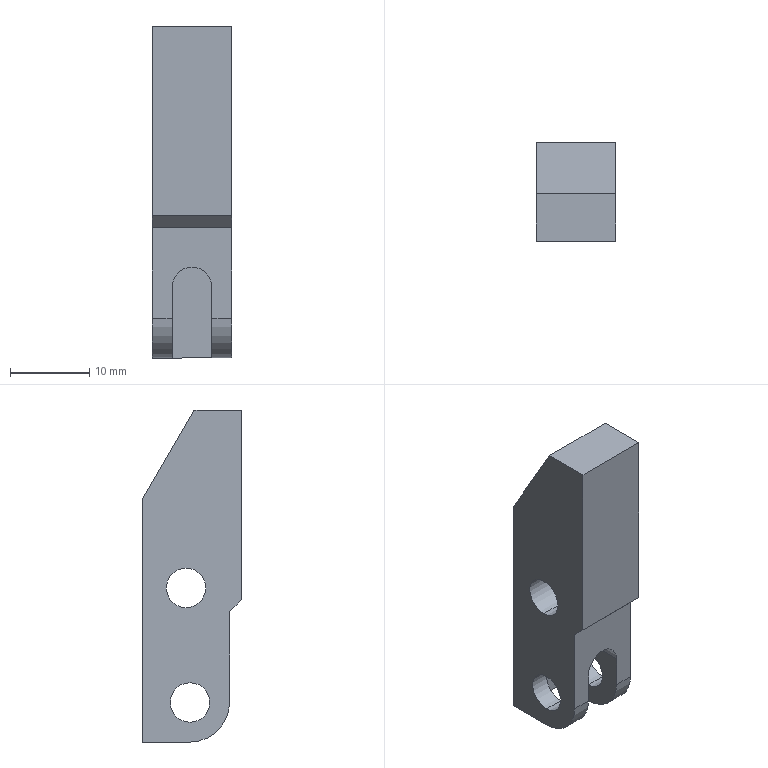Component | SolidWorks | LeverHydraulicRod22-1_HLKA-22_-1-1 | 1 solid | 21 faces | box 10 x 12.5 x 42 mm | volume 3756 mm3 | plane 12 | cylinder 9 | commonest cylinder face diameters 5 x7 10 x2
STEP:
#1=COLOUR_RGB('',0.7922,0.8196,0.9333);
#2=FILL_AREA_STYLE_COLOUR('',#1);
#3=FILL_AREA_STYLE('',(#2));
#4=SURFACE_STYLE_FILL_AREA(#3);
#5=SURFACE_SIDE_STYLE('',(#4));
#6=SURFACE_STYLE_USAGE(.BOTH.,#5);
#7=PRESENTATION_STYLE_ASSIGNMENT((#6));
#8=CARTESIAN_POINT('',(-2.465,4.49,-3.15));
#9=VERTEX_POINT('',#8);
#10=CARTESIAN_POINT('',(-2.465,4.49,-2.953));
#11=VERTEX_POINT('',#10);
#12=CARTESIAN_POINT('',(-2.465,4.49,-3.051));
#13=DIRECTION('',(-1.,-0.,-0.));
#14=DIRECTION('',(0.,0.,1.));
#15=AXIS2_PLACEMENT_3D('',#12,#13,#14);
#16=CIRCLE('',#15,0.09843);
#17=EDGE_CURVE('',#9,#11,#16,.T.);
#18=ORIENTED_EDGE('',*,*,#17,.F.);
#19=CARTESIAN_POINT('',(-2.859,4.49,-3.15));
#20=VERTEX_POINT('',#19);
#21=CARTESIAN_POINT('',(-2.387,4.49,-3.15));
#22=DIRECTION('',(-1.,-0.,-0.));
#23=VECTOR('',#22,39.37);
#24=LINE('',#21,#23);
#25=EDGE_CURVE('',#9,#20,#24,.T.);
#26=ORIENTED_EDGE('',*,*,#25,.T.);
#27=CARTESIAN_POINT('',(-2.859,4.49,-2.953));
#28=VERTEX_POINT('',#27);
#29=CARTESIAN_POINT('',(-2.859,4.49,-3.051));
#30=DIRECTION('',(-1.,-0.,-0.));
#31=DIRECTION('',(0.,0.,1.));
#32=AXIS2_PLACEMENT_3D('',#29,#30,#31);
#33=CIRCLE('',#32,0.09843);
#34=EDGE_CURVE('',#20,#28,#33,.T.);
#35=ORIENTED_EDGE('',*,*,#34,.T.);
#36=CARTESIAN_POINT('',(-2.387,4.49,-2.953));
#37=DIRECTION('',(-1.,-0.,-0.));
#38=VECTOR('',#37,39.37);
#39=LINE('',#36,#38);
#40=EDGE_CURVE('',#11,#28,#39,.T.);
#41=ORIENTED_EDGE('',*,*,#40,.F.);
#42=EDGE_LOOP('',(#18,#26,#35,#41));
#43=FACE_OUTER_BOUND('',#42,.T.);
#44=CARTESIAN_POINT('',(-2.387,4.49,-3.051));
#45=DIRECTION('',(-1.,-0.,-0.));
#46=DIRECTION('',(-0.,0.,1.));
#47=AXIS2_PLACEMENT_3D('',#44,#45,#46);
#48=CYLINDRICAL_SURFACE('',#47,0.09843);
#49=ADVANCED_FACE('',(#43),#48,.F.);
#50=CARTESIAN_POINT('',(-2.465,4.47,-3.72));
#51=VERTEX_POINT('',#50);
#52=CARTESIAN_POINT('',(-2.465,4.47,-3.524));
#53=VERTEX_POINT('',#52);
#54=CARTESIAN_POINT('',(-2.465,4.47,-3.622));
#55=DIRECTION('',(-1.,-0.,-0.));
#56=DIRECTION('',(0.,0.,1.));
#57=AXIS2_PLACEMENT_3D('',#54,#55,#56);
#58=CIRCLE('',#57,0.09843);
#59=EDGE_CURVE('',#51,#53,#58,.T.);
#60=ORIENTED_EDGE('',*,*,#59,.F.);
#61=CARTESIAN_POINT('',(-2.564,4.47,-3.72));
#62=VERTEX_POINT('',#61);
#63=CARTESIAN_POINT('',(-2.387,4.47,-3.72));
#64=DIRECTION('',(-1.,-0.,-0.));
#65=VECTOR('',#64,39.37);
#66=LINE('',#63,#65);
#67=EDGE_CURVE('',#51,#62,#66,.T.);
#68=ORIENTED_EDGE('',*,*,#67,.T.);
#69=CARTESIAN_POINT('',(-2.564,4.47,-3.524));
#70=VERTEX_POINT('',#69);
#71=CARTESIAN_POINT('',(-2.564,4.47,-3.622));
#72=DIRECTION('',(-1.,-0.,-0.));
#73=DIRECTION('',(0.,0.,-1.));
#74=AXIS2_PLACEMENT_3D('',#71,#72,#73);
#75=CIRCLE('',#74,0.09843);
#76=EDGE_CURVE('',#62,#70,#75,.T.);
#77=ORIENTED_EDGE('',*,*,#76,.T.);
#78=CARTESIAN_POINT('',(-2.387,4.47,-3.524));
#79=DIRECTION('',(-1.,-0.,-0.));
#80=VECTOR('',#79,39.37);
#81=LINE('',#78,#80);
#82=EDGE_CURVE('',#53,#70,#81,.T.);
#83=ORIENTED_EDGE('',*,*,#82,.F.);
#84=EDGE_LOOP('',(#60,#68,#77,#83));
#85=FACE_OUTER_BOUND('',#84,.T.);
#86=CARTESIAN_POINT('',(-2.387,4.47,-3.622));
#87=DIRECTION('',(-1.,-0.,-0.));
#88=DIRECTION('',(-0.,0.,1.));
#89=AXIS2_PLACEMENT_3D('',#86,#87,#88);
#90=CYLINDRICAL_SURFACE('',#89,0.09843);
#91=ADVANCED_FACE('',(#85),#90,.F.);
#92=CARTESIAN_POINT('',(-2.761,4.47,-3.524));
#93=VERTEX_POINT('',#92);
#94=CARTESIAN_POINT('',(-2.761,4.47,-3.72));
#95=VERTEX_POINT('',#94);
#96=CARTESIAN_POINT('',(-2.761,4.47,-3.622));
#97=DIRECTION('',(1.,0.,0.));
#98=DIRECTION('',(0.,0.,1.));
#99=AXIS2_PLACEMENT_3D('',#96,#97,#98);
#100=CIRCLE('',#99,0.09843);
#101=EDGE_CURVE('',#93,#95,#100,.T.);
#102=ORIENTED_EDGE('',*,*,#101,.T.);
#103=CARTESIAN_POINT('',(-2.859,4.47,-3.72));
#104=VERTEX_POINT('',#103);
#105=CARTESIAN_POINT('',(-2.387,4.47,-3.72));
#106=DIRECTION('',(-1.,-0.,-0.));
#107=VECTOR('',#106,39.37);
#108=LINE('',#105,#107);
#109=EDGE_CURVE('',#95,#104,#108,.T.);
#110=ORIENTED_EDGE('',*,*,#109,.T.);
#111=CARTESIAN_POINT('',(-2.859,4.47,-3.524));
#112=VERTEX_POINT('',#111);
#113=CARTESIAN_POINT('',(-2.859,4.47,-3.622));
#114=DIRECTION('',(-1.,-0.,-0.));
#115=DIRECTION('',(0.,0.,1.));
#116=AXIS2_PLACEMENT_3D('',#113,#114,#115);
#117=CIRCLE('',#116,0.09843);
#118=EDGE_CURVE('',#104,#112,#117,.T.);
#119=ORIENTED_EDGE('',*,*,#118,.T.);
#120=CARTESIAN_POINT('',(-2.387,4.47,-3.524));
#121=DIRECTION('',(-1.,-0.,-0.));
#122=VECTOR('',#121,39.37);
#123=LINE('',#120,#122);
#124=EDGE_CURVE('',#93,#112,#123,.T.);
#125=ORIENTED_EDGE('',*,*,#124,.F.);
#126=EDGE_LOOP('',(#102,#110,#119,#125));
#127=FACE_OUTER_BOUND('',#126,.T.);
#128=CARTESIAN_POINT('',(-2.387,4.47,-3.622));
#129=DIRECTION('',(-1.,-0.,-0.));
#130=DIRECTION('',(-0.,0.,1.));
#131=AXIS2_PLACEMENT_3D('',#128,#129,#130);
#132=CYLINDRICAL_SURFACE('',#131,0.09843);
#133=ADVANCED_FACE('',(#127),#132,.F.);
#134=CARTESIAN_POINT('',(-2.761,4.274,-3.465));
#135=VERTEX_POINT('',#134);
#136=CARTESIAN_POINT('',(-2.761,4.274,-3.622));
#137=VERTEX_POINT('',#136);
#138=CARTESIAN_POINT('',(-2.761,4.274,-3.914));
#139=DIRECTION('',(0.,-0.,-1.));
#140=VECTOR('',#139,39.37);
#141=LINE('',#138,#140);
#142=EDGE_CURVE('',#135,#137,#141,.T.);
#143=ORIENTED_EDGE('',*,*,#142,.F.);
#144=CARTESIAN_POINT('',(-2.564,4.274,-3.465));
#145=VERTEX_POINT('',#144);
#146=CARTESIAN_POINT('',(-2.662,4.274,-3.465));
#147=DIRECTION('',(-0.,-1.,0.));
#148=DIRECTION('',(-1.,0.,0.));
#149=AXIS2_PLACEMENT_3D('',#146,#147,#148);
#150=CIRCLE('',#149,0.09843);
#151=EDGE_CURVE('',#145,#135,#150,.T.);
#152=ORIENTED_EDGE('',*,*,#151,.F.);
#153=CARTESIAN_POINT('',(-2.564,4.274,-3.622));
#154=VERTEX_POINT('',#153);
#155=CARTESIAN_POINT('',(-2.564,4.274,-3.914));
#156=DIRECTION('',(-0.,0.,1.));
#157=VECTOR('',#156,39.37);
#158=LINE('',#155,#157);
#159=EDGE_CURVE('',#154,#145,#158,.T.);
#160=ORIENTED_EDGE('',*,*,#159,.F.);
#161=CARTESIAN_POINT('',(-2.465,4.274,-3.622));
#162=VERTEX_POINT('',#161);
#163=CARTESIAN_POINT('',(-2.859,4.274,-3.622));
#164=DIRECTION('',(1.,0.,0.));
#165=VECTOR('',#164,39.37);
#166=LINE('',#163,#165);
#167=EDGE_CURVE('',#154,#162,#166,.T.);
#168=ORIENTED_EDGE('',*,*,#167,.T.);
#169=CARTESIAN_POINT('',(-2.465,4.274,-3.169));
#170=VERTEX_POINT('',#169);
#171=CARTESIAN_POINT('',(-2.465,4.274,-3.819));
#172=DIRECTION('',(-0.,0.,1.));
#173=VECTOR('',#172,39.37);
#174=LINE('',#171,#173);
#175=EDGE_CURVE('',#162,#170,#174,.T.);
#176=ORIENTED_EDGE('',*,*,#175,.T.);
#177=CARTESIAN_POINT('',(-2.859,4.274,-3.169));
#178=VERTEX_POINT('',#177);
#179=CARTESIAN_POINT('',(-2.859,4.274,-3.169));
#180=DIRECTION('',(1.,0.,0.));
#181=VECTOR('',#180,39.37);
#182=LINE('',#179,#181);
#183=EDGE_CURVE('',#178,#170,#182,.T.);
#184=ORIENTED_EDGE('',*,*,#183,.F.);
#185=CARTESIAN_POINT('',(-2.859,4.274,-3.622));
#186=VERTEX_POINT('',#185);
#187=CARTESIAN_POINT('',(-2.859,4.274,-3.819));
#188=DIRECTION('',(-0.,0.,1.));
#189=VECTOR('',#188,39.37);
#190=LINE('',#187,#189);
#191=EDGE_CURVE('',#186,#178,#190,.T.);
#192=ORIENTED_EDGE('',*,*,#191,.F.);
#193=CARTESIAN_POINT('',(-2.859,4.274,-3.622));
#194=DIRECTION('',(1.,0.,0.));
#195=VECTOR('',#194,39.37);
#196=LINE('',#193,#195);
#197=EDGE_CURVE('',#186,#137,#196,.T.);
#198=ORIENTED_EDGE('',*,*,#197,.T.);
#199=EDGE_LOOP('',(#143,#152,#160,#168,#176,#184,#192,#198));
#200=FACE_OUTER_BOUND('',#199,.T.);
#201=CARTESIAN_POINT('',(-2.859,4.274,-3.819));
#202=DIRECTION('',(0.,1.,-0.));
#203=DIRECTION('',(-0.,0.,1.));
#204=AXIS2_PLACEMENT_3D('',#201,#202,#203);
#205=PLANE('',#204);
#206=ADVANCED_FACE('',(#200),#205,.F.);
#207=CARTESIAN_POINT('',(-2.859,4.47,-3.819));
#208=VERTEX_POINT('',#207);
#209=CARTESIAN_POINT('',(-2.859,4.47,-3.622));
#210=DIRECTION('',(-1.,-0.,-0.));
#211=DIRECTION('',(-0.,0.,1.));
#212=AXIS2_PLACEMENT_3D('',#209,#210,#211);
#213=CIRCLE('',#212,0.1969);
#214=EDGE_CURVE('',#208,#186,#213,.T.);
#215=ORIENTED_EDGE('',*,*,#214,.F.);
#216=CARTESIAN_POINT('',(-2.761,4.47,-3.819));
#217=VERTEX_POINT('',#216);
#218=CARTESIAN_POINT('',(-2.859,4.47,-3.819));
#219=DIRECTION('',(-1.,-0.,-0.));
#220=VECTOR('',#219,39.37);
#221=LINE('',#218,#220);
#222=EDGE_CURVE('',#217,#208,#221,.T.);
#223=ORIENTED_EDGE('',*,*,#222,.F.);
#224=CARTESIAN_POINT('',(-2.761,4.47,-3.622));
#225=DIRECTION('',(1.,0.,0.));
#226=DIRECTION('',(-0.,0.,1.));
#227=AXIS2_PLACEMENT_3D('',#224,#225,#226);
#228=CIRCLE('',#227,0.1969);
#229=EDGE_CURVE('',#137,#217,#228,.T.);
#230=ORIENTED_EDGE('',*,*,#229,.F.);
#231=ORIENTED_EDGE('',*,*,#197,.F.);
#232=EDGE_LOOP('',(#215,#223,#230,#231));
#233=FACE_OUTER_BOUND('',#232,.T.);
#234=CARTESIAN_POINT('',(-2.859,4.47,-3.622));
#235=DIRECTION('',(1.,0.,0.));
#236=DIRECTION('',(0.,0.,-1.));
#237=AXIS2_PLACEMENT_3D('',#234,#235,#236);
#238=CYLINDRICAL_SURFACE('',#237,0.1969);
#239=ADVANCED_FACE('',(#233),#238,.T.);
#240=CARTESIAN_POINT('',(-2.564,4.47,-3.819));
#241=VERTEX_POINT('',#240);
#242=CARTESIAN_POINT('',(-2.564,4.47,-3.622));
#243=DIRECTION('',(-1.,-0.,-0.));
#244=DIRECTION('',(0.,0.,-1.));
#245=AXIS2_PLACEMENT_3D('',#242,#243,#244);
#246=CIRCLE('',#245,0.1969);
#247=EDGE_CURVE('',#241,#154,#246,.T.);
#248=ORIENTED_EDGE('',*,*,#247,.F.);
#249=CARTESIAN_POINT('',(-2.465,4.47,-3.819));
#250=VERTEX_POINT('',#249);
#251=CARTESIAN_POINT('',(-2.859,4.47,-3.819));
#252=DIRECTION('',(-1.,-0.,-0.));
#253=VECTOR('',#252,39.37);
#254=LINE('',#251,#253);
#255=EDGE_CURVE('',#250,#241,#254,.T.);
#256=ORIENTED_EDGE('',*,*,#255,.F.);
#257=CARTESIAN_POINT('',(-2.465,4.47,-3.622));
#258=DIRECTION('',(1.,0.,0.));
#259=DIRECTION('',(-0.,0.,1.));
#260=AXIS2_PLACEMENT_3D('',#257,#258,#259);
#261=CIRCLE('',#260,0.1969);
#262=EDGE_CURVE('',#162,#250,#261,.T.);
#263=ORIENTED_EDGE('',*,*,#262,.F.);
#264=ORIENTED_EDGE('',*,*,#167,.F.);
#265=EDGE_LOOP('',(#248,#256,#263,#264));
#266=FACE_OUTER_BOUND('',#265,.T.);
#267=CARTESIAN_POINT('',(-2.859,4.47,-3.622));
#268=DIRECTION('',(1.,0.,0.));
#269=DIRECTION('',(0.,0.,-1.));
#270=AXIS2_PLACEMENT_3D('',#267,#268,#269);
#271=CYLINDRICAL_SURFACE('',#270,0.1969);
#272=ADVANCED_FACE('',(#266),#271,.T.);
#273=CARTESIAN_POINT('',(-2.564,4.667,-3.465));
#274=VERTEX_POINT('',#273);
#275=CARTESIAN_POINT('',(-2.564,4.667,-3.465));
#276=DIRECTION('',(-0.,-1.,0.));
#277=VECTOR('',#276,39.37);
#278=LINE('',#275,#277);
#279=EDGE_CURVE('',#274,#145,#278,.T.);
#280=ORIENTED_EDGE('',*,*,#279,.F.);
#281=CARTESIAN_POINT('',(-2.564,4.667,-3.819));
#282=VERTEX_POINT('',#281);
#283=CARTESIAN_POINT('',(-2.564,4.667,-3.914));
#284=DIRECTION('',(-0.,0.,1.));
#285=VECTOR('',#284,39.37);
#286=LINE('',#283,#285);
#287=EDGE_CURVE('',#282,#274,#286,.T.);
#288=ORIENTED_EDGE('',*,*,#287,.F.);
#289=CARTESIAN_POINT('',(-2.564,4.707,-3.819));
#290=DIRECTION('',(0.,1.,-0.));
#291=VECTOR('',#290,39.37);
#292=LINE('',#289,#291);
#293=EDGE_CURVE('',#241,#282,#292,.T.);
#294=ORIENTED_EDGE('',*,*,#293,.F.);
#295=ORIENTED_EDGE('',*,*,#247,.T.);
#296=ORIENTED_EDGE('',*,*,#159,.T.);
#297=EDGE_LOOP('',(#280,#288,#294,#295,#296));
#298=FACE_OUTER_BOUND('',#297,.T.);
#299=CARTESIAN_POINT('',(-2.564,4.47,-3.622));
#300=DIRECTION('',(-1.,-0.,-0.));
#301=DIRECTION('',(0.,0.,-1.));
#302=AXIS2_PLACEMENT_3D('',#299,#300,#301);
#303=CIRCLE('',#302,0.09843);
#304=EDGE_CURVE('',#70,#62,#303,.T.);
#305=ORIENTED_EDGE('',*,*,#304,.F.);
#306=ORIENTED_EDGE('',*,*,#76,.F.);
#307=EDGE_LOOP('',(#305,#306));
#308=FACE_BOUND('',#307,.T.);
#309=CARTESIAN_POINT('',(-2.564,4.667,-3.914));
#310=DIRECTION('',(1.,0.,0.));
#311=DIRECTION('',(-0.,-1.,0.));
#312=AXIS2_PLACEMENT_3D('',#309,#310,#311);
#313=PLANE('',#312);
#314=ADVANCED_FACE('',(#298,#308),#313,.F.);
#315=ORIENTED_EDGE('',*,*,#101,.F.);
#316=CARTESIAN_POINT('',(-2.761,4.47,-3.622));
#317=DIRECTION('',(1.,0.,0.));
#318=DIRECTION('',(0.,0.,1.));
#319=AXIS2_PLACEMENT_3D('',#316,#317,#318);
#320=CIRCLE('',#319,0.09843);
#321=EDGE_CURVE('',#95,#93,#320,.T.);
#322=ORIENTED_EDGE('',*,*,#321,.F.);
#323=EDGE_LOOP('',(#315,#322));
#324=FACE_BOUND('',#323,.T.);
#325=CARTESIAN_POINT('',(-2.761,4.667,-3.819));
#326=VERTEX_POINT('',#325);
#327=CARTESIAN_POINT('',(-2.761,4.707,-3.819));
#328=DIRECTION('',(-0.,-1.,0.));
#329=VECTOR('',#328,39.37);
#330=LINE('',#327,#329);
#331=EDGE_CURVE('',#326,#217,#330,.T.);
#332=ORIENTED_EDGE('',*,*,#331,.F.);
#333=CARTESIAN_POINT('',(-2.761,4.667,-3.465));
#334=VERTEX_POINT('',#333);
#335=CARTESIAN_POINT('',(-2.761,4.667,-3.914));
#336=DIRECTION('',(0.,-0.,-1.));
#337=VECTOR('',#336,39.37);
#338=LINE('',#335,#337);
#339=EDGE_CURVE('',#334,#326,#338,.T.);
#340=ORIENTED_EDGE('',*,*,#339,.F.);
#341=CARTESIAN_POINT('',(-2.761,4.667,-3.465));
#342=DIRECTION('',(-0.,-1.,0.));
#343=VECTOR('',#342,39.37);
#344=LINE('',#341,#343);
#345=EDGE_CURVE('',#334,#135,#344,.T.);
#346=ORIENTED_EDGE('',*,*,#345,.T.);
#347=ORIENTED_EDGE('',*,*,#142,.T.);
#348=ORIENTED_EDGE('',*,*,#229,.T.);
#349=EDGE_LOOP('',(#332,#340,#346,#347,#348));
#350=FACE_OUTER_BOUND('',#349,.T.);
#351=CARTESIAN_POINT('',(-2.761,4.667,-3.914));
#352=DIRECTION('',(-1.,-0.,-0.));
#353=DIRECTION('',(-0.,0.,1.));
#354=AXIS2_PLACEMENT_3D('',#351,#352,#353);
#355=PLANE('',#354);
#356=ADVANCED_FACE('',(#324,#350),#355,.F.);
#357=ORIENTED_EDGE('',*,*,#339,.T.);
#358=CARTESIAN_POINT('',(-2.859,4.667,-3.819));
#359=DIRECTION('',(1.,0.,0.));
#360=VECTOR('',#359,39.37);
#361=LINE('',#358,#360);
#362=EDGE_CURVE('',#326,#282,#361,.T.);
#363=ORIENTED_EDGE('',*,*,#362,.T.);
#364=ORIENTED_EDGE('',*,*,#287,.T.);
#365=CARTESIAN_POINT('',(-2.662,4.667,-3.465));
#366=DIRECTION('',(0.,1.,-0.));
#367=DIRECTION('',(1.,0.,0.));
#368=AXIS2_PLACEMENT_3D('',#365,#366,#367);
#369=CIRCLE('',#368,0.09843);
#370=EDGE_CURVE('',#334,#274,#369,.T.);
#371=ORIENTED_EDGE('',*,*,#370,.F.);
#372=EDGE_LOOP('',(#357,#363,#364,#371));
#373=FACE_OUTER_BOUND('',#372,.T.);
#374=CARTESIAN_POINT('',(-2.662,4.667,-3.484));
#375=DIRECTION('',(-0.,-1.,0.));
#376=DIRECTION('',(1.,0.,0.));
#377=AXIS2_PLACEMENT_3D('',#374,#375,#376);
#378=PLANE('',#377);
#379=ADVANCED_FACE('',(#373),#378,.T.);
#380=CARTESIAN_POINT('',(-2.465,4.47,-3.622));
#381=DIRECTION('',(-1.,-0.,-0.));
#382=DIRECTION('',(0.,0.,1.));
#383=AXIS2_PLACEMENT_3D('',#380,#381,#382);
#384=CIRCLE('',#383,0.09843);
#385=EDGE_CURVE('',#53,#51,#384,.T.);
#386=ORIENTED_EDGE('',*,*,#385,.T.);
#387=ORIENTED_EDGE('',*,*,#59,.T.);
#388=EDGE_LOOP('',(#386,#387));
#389=FACE_BOUND('',#388,.T.);
#390=CARTESIAN_POINT('',(-2.465,4.49,-3.051));
#391=DIRECTION('',(-1.,-0.,-0.));
#392=DIRECTION('',(0.,0.,1.));
#393=AXIS2_PLACEMENT_3D('',#390,#391,#392);
#394=CIRCLE('',#393,0.09843);
#395=EDGE_CURVE('',#11,#9,#394,.T.);
#396=ORIENTED_EDGE('',*,*,#395,.T.);
#397=ORIENTED_EDGE('',*,*,#17,.T.);
#398=EDGE_LOOP('',(#396,#397));
#399=FACE_BOUND('',#398,.T.);
#400=ORIENTED_EDGE('',*,*,#175,.F.);
#401=ORIENTED_EDGE('',*,*,#262,.T.);
#402=CARTESIAN_POINT('',(-2.465,4.707,-3.819));
#403=VERTEX_POINT('',#402);
#404=CARTESIAN_POINT('',(-2.465,4.707,-3.819));
#405=DIRECTION('',(-0.,-1.,0.));
#406=VECTOR('',#405,39.37);
#407=LINE('',#404,#406);
#408=EDGE_CURVE('',#403,#250,#407,.T.);
#409=ORIENTED_EDGE('',*,*,#408,.F.);
#410=CARTESIAN_POINT('',(-2.465,4.707,-2.609));
#411=VERTEX_POINT('',#410);
#412=CARTESIAN_POINT('',(-2.465,4.707,-2.609));
#413=DIRECTION('',(0.,-0.,-1.));
#414=VECTOR('',#413,39.37);
#415=LINE('',#412,#414);
#416=EDGE_CURVE('',#411,#403,#415,.T.);
#417=ORIENTED_EDGE('',*,*,#416,.F.);
#418=CARTESIAN_POINT('',(-2.465,4.451,-2.165));
#419=VERTEX_POINT('',#418);
#420=CARTESIAN_POINT('',(-2.465,4.451,-2.165));
#421=DIRECTION('',(0.,0.5,-0.866));
#422=VECTOR('',#421,39.37);
#423=LINE('',#420,#422);
#424=EDGE_CURVE('',#419,#411,#423,.T.);
#425=ORIENTED_EDGE('',*,*,#424,.F.);
#426=CARTESIAN_POINT('',(-2.465,4.214,-2.165));
#427=VERTEX_POINT('',#426);
#428=CARTESIAN_POINT('',(-2.465,4.214,-2.165));
#429=DIRECTION('',(0.,1.,-0.));
#430=VECTOR('',#429,39.37);
#431=LINE('',#428,#430);
#432=EDGE_CURVE('',#427,#419,#431,.T.);
#433=ORIENTED_EDGE('',*,*,#432,.F.);
#434=CARTESIAN_POINT('',(-2.465,4.214,-3.11));
#435=VERTEX_POINT('',#434);
#436=CARTESIAN_POINT('',(-2.465,4.214,-3.11));
#437=DIRECTION('',(-0.,0.,1.));
#438=VECTOR('',#437,39.37);
#439=LINE('',#436,#438);
#440=EDGE_CURVE('',#435,#427,#439,.T.);
#441=ORIENTED_EDGE('',*,*,#440,.F.);
#442=CARTESIAN_POINT('',(-2.465,4.274,-3.169));
#443=DIRECTION('',(-0.,-0.7071,0.7071));
#444=VECTOR('',#443,39.37);
#445=LINE('',#442,#444);
#446=EDGE_CURVE('',#170,#435,#445,.T.);
#447=ORIENTED_EDGE('',*,*,#446,.F.);
#448=EDGE_LOOP('',(#400,#401,#409,#417,#425,#433,#441,#447));
#449=FACE_OUTER_BOUND('',#448,.T.);
#450=CARTESIAN_POINT('',(-2.465,4.274,-3.819));
#451=DIRECTION('',(-1.,-0.,-0.));
#452=DIRECTION('',(-0.,0.,1.));
#453=AXIS2_PLACEMENT_3D('',#450,#451,#452);
#454=PLANE('',#453);
#455=ADVANCED_FACE('',(#389,#399,#449),#454,.F.);
#456=CARTESIAN_POINT('',(-2.859,4.47,-3.622));
#457=DIRECTION('',(-1.,-0.,-0.));
#458=DIRECTION('',(0.,0.,1.));
#459=AXIS2_PLACEMENT_3D('',#456,#457,#458);
#460=CIRCLE('',#459,0.09843);
#461=EDGE_CURVE('',#112,#104,#460,.T.);
#462=ORIENTED_EDGE('',*,*,#461,.F.);
#463=ORIENTED_EDGE('',*,*,#118,.F.);
#464=EDGE_LOOP('',(#462,#463));
#465=FACE_BOUND('',#464,.T.);
#466=CARTESIAN_POINT('',(-2.859,4.49,-3.051));
#467=DIRECTION('',(-1.,-0.,-0.));
#468=DIRECTION('',(0.,0.,1.));
#469=AXIS2_PLACEMENT_3D('',#466,#467,#468);
#470=CIRCLE('',#469,0.09843);
#471=EDGE_CURVE('',#28,#20,#470,.T.);
#472=ORIENTED_EDGE('',*,*,#471,.F.);
#473=ORIENTED_EDGE('',*,*,#34,.F.);
#474=EDGE_LOOP('',(#472,#473));
#475=FACE_BOUND('',#474,.T.);
#476=CARTESIAN_POINT('',(-2.859,4.707,-3.819));
#477=VERTEX_POINT('',#476);
#478=CARTESIAN_POINT('',(-2.859,4.707,-3.819));
#479=DIRECTION('',(-0.,-1.,0.));
#480=VECTOR('',#479,39.37);
#481=LINE('',#478,#480);
#482=EDGE_CURVE('',#477,#208,#481,.T.);
#483=ORIENTED_EDGE('',*,*,#482,.T.);
#484=ORIENTED_EDGE('',*,*,#214,.T.);
#485=ORIENTED_EDGE('',*,*,#191,.T.);
#486=CARTESIAN_POINT('',(-2.859,4.214,-3.11));
#487=VERTEX_POINT('',#486);
#488=CARTESIAN_POINT('',(-2.859,4.274,-3.169));
#489=DIRECTION('',(-0.,-0.7071,0.7071));
#490=VECTOR('',#489,39.37);
#491=LINE('',#488,#490);
#492=EDGE_CURVE('',#178,#487,#491,.T.);
#493=ORIENTED_EDGE('',*,*,#492,.T.);
#494=CARTESIAN_POINT('',(-2.859,4.214,-2.165));
#495=VERTEX_POINT('',#494);
#496=CARTESIAN_POINT('',(-2.859,4.214,-3.11));
#497=DIRECTION('',(-0.,0.,1.));
#498=VECTOR('',#497,39.37);
#499=LINE('',#496,#498);
#500=EDGE_CURVE('',#487,#495,#499,.T.);
#501=ORIENTED_EDGE('',*,*,#500,.T.);
#502=CARTESIAN_POINT('',(-2.859,4.451,-2.165));
#503=VERTEX_POINT('',#502);
#504=CARTESIAN_POINT('',(-2.859,4.214,-2.165));
#505=DIRECTION('',(0.,1.,-0.));
#506=VECTOR('',#505,39.37);
#507=LINE('',#504,#506);
#508=EDGE_CURVE('',#495,#503,#507,.T.);
#509=ORIENTED_EDGE('',*,*,#508,.T.);
#510=CARTESIAN_POINT('',(-2.859,4.707,-2.609));
#511=VERTEX_POINT('',#510);
#512=CARTESIAN_POINT('',(-2.859,4.451,-2.165));
#513=DIRECTION('',(0.,0.5,-0.866));
#514=VECTOR('',#513,39.37);
#515=LINE('',#512,#514);
#516=EDGE_CURVE('',#503,#511,#515,.T.);
#517=ORIENTED_EDGE('',*,*,#516,.T.);
#518=CARTESIAN_POINT('',(-2.859,4.707,-2.609));
#519=DIRECTION('',(0.,-0.,-1.));
#520=VECTOR('',#519,39.37);
#521=LINE('',#518,#520);
#522=EDGE_CURVE('',#511,#477,#521,.T.);
#523=ORIENTED_EDGE('',*,*,#522,.T.);
#524=EDGE_LOOP('',(#483,#484,#485,#493,#501,#509,#517,#523));
#525=FACE_OUTER_BOUND('',#524,.T.);
#526=CARTESIAN_POINT('',(-2.859,4.274,-3.819));
#527=DIRECTION('',(-1.,-0.,-0.));
#528=DIRECTION('',(-0.,0.,1.));
#529=AXIS2_PLACEMENT_3D('',#526,#527,#528);
#530=PLANE('',#529);
#531=ADVANCED_FACE('',(#465,#475,#525),#530,.T.);
#532=ORIENTED_EDGE('',*,*,#416,.T.);
#533=CARTESIAN_POINT('',(-2.859,4.707,-3.819));
#534=DIRECTION('',(1.,0.,0.));
#535=VECTOR('',#534,39.37);
#536=LINE('',#533,#535);
#537=EDGE_CURVE('',#477,#403,#536,.T.);
#538=ORIENTED_EDGE('',*,*,#537,.F.);
#539=ORIENTED_EDGE('',*,*,#522,.F.);
#540=CARTESIAN_POINT('',(-2.859,4.707,-2.609));
#541=DIRECTION('',(1.,0.,0.));
#542=VECTOR('',#541,39.37);
#543=LINE('',#540,#542);
#544=EDGE_CURVE('',#511,#411,#543,.T.);
#545=ORIENTED_EDGE('',*,*,#544,.T.);
#546=EDGE_LOOP('',(#532,#538,#539,#545));
#547=FACE_OUTER_BOUND('',#546,.T.);
#548=CARTESIAN_POINT('',(-2.859,4.707,-2.609));
#549=DIRECTION('',(-0.,-1.,0.));
#550=DIRECTION('',(1.,0.,0.));
#551=AXIS2_PLACEMENT_3D('',#548,#549,#550);
#552=PLANE('',#551);
#553=ADVANCED_FACE('',(#547),#552,.F.);
#554=ORIENTED_EDGE('',*,*,#424,.T.);
#555=ORIENTED_EDGE('',*,*,#544,.F.);
#556=ORIENTED_EDGE('',*,*,#516,.F.);
#557=CARTESIAN_POINT('',(-2.859,4.451,-2.165));
#558=DIRECTION('',(1.,0.,0.));
#559=VECTOR('',#558,39.37);
#560=LINE('',#557,#559);
#561=EDGE_CURVE('',#503,#419,#560,.T.);
#562=ORIENTED_EDGE('',*,*,#561,.T.);
#563=EDGE_LOOP('',(#554,#555,#556,#562));
#564=FACE_OUTER_BOUND('',#563,.T.);
#565=CARTESIAN_POINT('',(-2.859,4.451,-2.165));
#566=DIRECTION('',(0.,-0.866,-0.5));
#567=DIRECTION('',(0.,0.5,-0.866));
#568=AXIS2_PLACEMENT_3D('',#565,#566,#567);
#569=PLANE('',#568);
#570=ADVANCED_FACE('',(#564),#569,.F.);
#571=ORIENTED_EDGE('',*,*,#432,.T.);
#572=ORIENTED_EDGE('',*,*,#561,.F.);
#573=ORIENTED_EDGE('',*,*,#508,.F.);
#574=CARTESIAN_POINT('',(-2.859,4.214,-2.165));
#575=DIRECTION('',(1.,0.,0.));
#576=VECTOR('',#575,39.37);
#577=LINE('',#574,#576);
#578=EDGE_CURVE('',#495,#427,#577,.T.);
#579=ORIENTED_EDGE('',*,*,#578,.T.);
#580=EDGE_LOOP('',(#571,#572,#573,#579));
#581=FACE_OUTER_BOUND('',#580,.T.);
#582=CARTESIAN_POINT('',(-2.859,4.214,-2.165));
#583=DIRECTION('',(0.,-0.,-1.));
#584=DIRECTION('',(-1.,-0.,-0.));
#585=AXIS2_PLACEMENT_3D('',#582,#583,#584);
#586=PLANE('',#585);
#587=ADVANCED_FACE('',(#581),#586,.F.);
#588=ORIENTED_EDGE('',*,*,#440,.T.);
#589=ORIENTED_EDGE('',*,*,#578,.F.);
#590=ORIENTED_EDGE('',*,*,#500,.F.);
#591=CARTESIAN_POINT('',(-2.859,4.214,-3.11));
#592=DIRECTION('',(1.,0.,0.));
#593=VECTOR('',#592,39.37);
#594=LINE('',#591,#593);
#595=EDGE_CURVE('',#487,#435,#594,.T.);
#596=ORIENTED_EDGE('',*,*,#595,.T.);
#597=EDGE_LOOP('',(#588,#589,#590,#596));
#598=FACE_OUTER_BOUND('',#597,.T.);
#599=CARTESIAN_POINT('',(-2.859,4.214,-3.11));
#600=DIRECTION('',(-0.,1.,-0.));
#601=DIRECTION('',(-0.,0.,1.));
#602=AXIS2_PLACEMENT_3D('',#599,#600,#601);
#603=PLANE('',#602);
#604=ADVANCED_FACE('',(#598),#603,.F.);
#605=ORIENTED_EDGE('',*,*,#446,.T.);
#606=ORIENTED_EDGE('',*,*,#595,.F.);
#607=ORIENTED_EDGE('',*,*,#492,.F.);
#608=ORIENTED_EDGE('',*,*,#183,.T.);
#609=EDGE_LOOP('',(#605,#606,#607,#608));
#610=FACE_OUTER_BOUND('',#609,.T.);
#611=CARTESIAN_POINT('',(-2.859,4.274,-3.169));
#612=DIRECTION('',(-0.,0.7071,0.7071));
#613=DIRECTION('',(1.,0.,0.));
#614=AXIS2_PLACEMENT_3D('',#611,#612,#613);
#615=PLANE('',#614);
#616=ADVANCED_FACE('',(#610),#615,.F.);
#617=ORIENTED_EDGE('',*,*,#408,.T.);
#618=ORIENTED_EDGE('',*,*,#255,.T.);
#619=ORIENTED_EDGE('',*,*,#293,.T.);
#620=ORIENTED_EDGE('',*,*,#362,.F.);
#621=ORIENTED_EDGE('',*,*,#331,.T.);
#622=ORIENTED_EDGE('',*,*,#222,.T.);
#623=ORIENTED_EDGE('',*,*,#482,.F.);
#624=ORIENTED_EDGE('',*,*,#537,.T.);
#625=EDGE_LOOP('',(#617,#618,#619,#620,#621,#622,#623,#624));
#626=FACE_OUTER_BOUND('',#625,.T.);
#627=CARTESIAN_POINT('',(-2.859,4.707,-3.819));
#628=DIRECTION('',(-0.,0.,1.));
#629=DIRECTION('',(0.,1.,-0.));
#630=AXIS2_PLACEMENT_3D('',#627,#628,#629);
#631=PLANE('',#630);
#632=ADVANCED_FACE('',(#626),#631,.F.);
#633=ORIENTED_EDGE('',*,*,#109,.F.);
#634=ORIENTED_EDGE('',*,*,#321,.T.);
#635=ORIENTED_EDGE('',*,*,#124,.T.);
#636=ORIENTED_EDGE('',*,*,#461,.T.);
#637=EDGE_LOOP('',(#633,#634,#635,#636));
#638=FACE_OUTER_BOUND('',#637,.T.);
#639=CARTESIAN_POINT('',(-2.387,4.47,-3.622));
#640=DIRECTION('',(-1.,-0.,-0.));
#641=DIRECTION('',(-0.,0.,1.));
#642=AXIS2_PLACEMENT_3D('',#639,#640,#641);
#643=CYLINDRICAL_SURFACE('',#642,0.09843);
#644=ADVANCED_FACE('',(#638),#643,.F.);
#645=ORIENTED_EDGE('',*,*,#67,.F.);
#646=ORIENTED_EDGE('',*,*,#385,.F.);
#647=ORIENTED_EDGE('',*,*,#82,.T.);
#648=ORIENTED_EDGE('',*,*,#304,.T.);
#649=EDGE_LOOP('',(#645,#646,#647,#648));
#650=FACE_OUTER_BOUND('',#649,.T.);
#651=CARTESIAN_POINT('',(-2.387,4.47,-3.622));
#652=DIRECTION('',(-1.,-0.,-0.));
#653=DIRECTION('',(-0.,0.,1.));
#654=AXIS2_PLACEMENT_3D('',#651,#652,#653);
#655=CYLINDRICAL_SURFACE('',#654,0.09843);
#656=ADVANCED_FACE('',(#650),#655,.F.);
#657=ORIENTED_EDGE('',*,*,#25,.F.);
#658=ORIENTED_EDGE('',*,*,#395,.F.);
#659=ORIENTED_EDGE('',*,*,#40,.T.);
#660=ORIENTED_EDGE('',*,*,#471,.T.);
#661=EDGE_LOOP('',(#657,#658,#659,#660));
#662=FACE_OUTER_BOUND('',#661,.T.);
#663=CARTESIAN_POINT('',(-2.387,4.49,-3.051));
#664=DIRECTION('',(-1.,-0.,-0.));
#665=DIRECTION('',(-0.,0.,1.));
#666=AXIS2_PLACEMENT_3D('',#663,#664,#665);
#667=CYLINDRICAL_SURFACE('',#666,0.09843);
#668=ADVANCED_FACE('',(#662),#667,.F.);
#669=ORIENTED_EDGE('',*,*,#151,.T.);
#670=ORIENTED_EDGE('',*,*,#345,.F.);
#671=ORIENTED_EDGE('',*,*,#370,.T.);
#672=ORIENTED_EDGE('',*,*,#279,.T.);
#673=EDGE_LOOP('',(#669,#670,#671,#672));
#674=FACE_OUTER_BOUND('',#673,.T.);
#675=CARTESIAN_POINT('',(-2.662,4.667,-3.465));
#676=DIRECTION('',(-0.,-1.,0.));
#677=DIRECTION('',(1.,0.,0.));
#678=AXIS2_PLACEMENT_3D('',#675,#676,#677);
#679=CYLINDRICAL_SURFACE('',#678,0.09843);
#680=ADVANCED_FACE('',(#674),#679,.F.);
#681=CLOSED_SHELL('',(#49,#91,#133,#206,#239,#272,#314,#356,#379,#455,#531,#553,#570,#587,#604,#616,#632,#644,#656,#668,#680));
#682=MANIFOLD_SOLID_BREP('',#681);
#683=STYLED_ITEM('',(#7),#682);
#684=PRESENTATION_LAYER_ASSIGNMENT('','',(#683));
#685=CARTESIAN_POINT('',(0.,0.,0.));
#686=DIRECTION('',(0.,0.,1.));
#687=DIRECTION('',(1.,0.,0.));
#688=AXIS2_PLACEMENT_3D('',#685,#686,#687);
#689=(LENGTH_UNIT()NAMED_UNIT(*)SI_UNIT($,.METRE.));
#690=LENGTH_MEASURE_WITH_UNIT(LENGTH_MEASURE(0.0254),#689);
#691=DIMENSIONAL_EXPONENTS(1.,0.,0.,0.,0.,0.,0.);
#692=(CONVERSION_BASED_UNIT('',#690)LENGTH_UNIT()NAMED_UNIT(#691));
#693=UNCERTAINTY_MEASURE_WITH_UNIT(LENGTH_MEASURE(0.00001),#692,'','');
#694=(NAMED_UNIT(*)PLANE_ANGLE_UNIT()SI_UNIT($,.RADIAN.));
#695=(NAMED_UNIT(*)SI_UNIT($,.STERADIAN.)SOLID_ANGLE_UNIT());
#696=(GEOMETRIC_REPRESENTATION_CONTEXT(3)GLOBAL_UNCERTAINTY_ASSIGNED_CONTEXT((#693))GLOBAL_UNIT_ASSIGNED_CONTEXT((#692,#694,#695))REPRESENTATION_CONTEXT('',''));
#697=ADVANCED_BREP_SHAPE_REPRESENTATION('',(#682,#688),#696);
#698=(LENGTH_UNIT()NAMED_UNIT(*)SI_UNIT($,.METRE.));
#699=LENGTH_MEASURE_WITH_UNIT(LENGTH_MEASURE(0.0254),#698);
#700=DIMENSIONAL_EXPONENTS(1.,0.,0.,0.,0.,0.,0.);
#701=(CONVERSION_BASED_UNIT('',#699)LENGTH_UNIT()NAMED_UNIT(#700));
#702=UNCERTAINTY_MEASURE_WITH_UNIT(LENGTH_MEASURE(0.00001),#701,'','');
#703=(NAMED_UNIT(*)PLANE_ANGLE_UNIT()SI_UNIT($,.RADIAN.));
#704=(NAMED_UNIT(*)SI_UNIT($,.STERADIAN.)SOLID_ANGLE_UNIT());
#705=(GEOMETRIC_REPRESENTATION_CONTEXT(3)GLOBAL_UNCERTAINTY_ASSIGNED_CONTEXT((#702))GLOBAL_UNIT_ASSIGNED_CONTEXT((#701,#703,#704))REPRESENTATION_CONTEXT('',''));
#706=MECHANICAL_DESIGN_GEOMETRIC_PRESENTATION_REPRESENTATION('',(#683),#705);